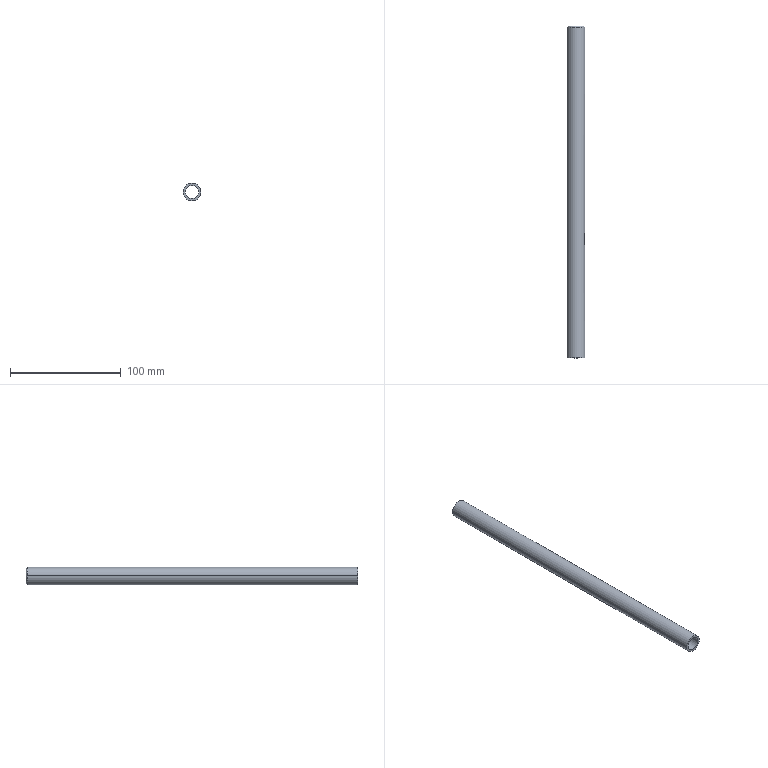Component | SolidWorks | GbgbMagnetPlacementTubeF8-1 | 1 solid | 11 faces | box 16 x 300 x 16 mm | volume 26347 mm3 | plane 5 | cylinder 4 | cone 2 | commonest cylinder face diameters 12 x2 16 x2
build123d program:
from build123d import *

# Parameters (mm, degrees)
SKETCH1_R           = 8
SKETCH1_R_2         = 6
BOSS_EXTRUDE1_DEPTH = 150
CHAMFER1_SIZE       = 1
SKETCH9_W           = 0.5
SKETCH9_H           = 10
CUT_EXTRUDE6_DEPTH  = 5


with BuildPart() as part:
    # Sketch1 → Boss-Extrude1 (new, symmetric)
    with BuildSketch(Plane(origin=(0, 0, 0), x_dir=(1, 0, 0), z_dir=(0, 1, 0))):
        with Locations(Location((0, 0, 0), (0, 0, 270))):
            Circle(SKETCH1_R)
        with Locations(Location((0, 0, 0), (0, 0, 270))):
            Circle(SKETCH1_R_2, mode=Mode.SUBTRACT)
    extrude(amount=BOSS_EXTRUDE1_DEPTH, both=True)

    # Chamfer1
    chamfer1_edges = [part.edges().sort_by_distance(p)[0] for p in [
        (0, -150, -8),
    ]]
    chamfer(chamfer1_edges, length=CHAMFER1_SIZE)

    # Sketch9 → Cut-Extrude6 (cut, symmetric)
    with BuildSketch(Plane(origin=(0, 0, 0), x_dir=(0, 0, -1), z_dir=(1, 0, 0))):
        with Locations((7.75, 42.5)):
            Rectangle(SKETCH9_W, SKETCH9_H)
    extrude(amount=CUT_EXTRUDE6_DEPTH, both=True, mode=Mode.SUBTRACT)


solid = part.part

# Placed as in the assembly
solid = solid.moved(Location((80.446, 537.34, 408.232), (180, -90, 0)))
STEP:
#1=COLOUR_RGB('',0.7922,0.8196,0.9333);
#2=FILL_AREA_STYLE_COLOUR('',#1);
#3=FILL_AREA_STYLE('',(#2));
#4=SURFACE_STYLE_FILL_AREA(#3);
#5=SURFACE_SIDE_STYLE('',(#4));
#6=SURFACE_STYLE_USAGE(.BOTH.,#5);
#7=PRESENTATION_STYLE_ASSIGNMENT((#6));
#8=CARTESIAN_POINT('',(3.443,27.061,16.072));
#9=VERTEX_POINT('',#8);
#10=CARTESIAN_POINT('',(2.892,27.061,16.072));
#11=VERTEX_POINT('',#10);
#12=CARTESIAN_POINT('',(3.167,27.061,16.072));
#13=DIRECTION('',(0.,1.,0.));
#14=DIRECTION('',(-1.,0.,0.));
#15=AXIS2_PLACEMENT_3D('',#12,#13,#14);
#16=CIRCLE('',#15,0.2756);
#17=EDGE_CURVE('',#9,#11,#16,.T.);
#18=ORIENTED_EDGE('',*,*,#17,.F.);
#19=CARTESIAN_POINT('',(3.482,27.021,16.072));
#20=VERTEX_POINT('',#19);
#21=CARTESIAN_POINT('',(3.482,27.021,16.072));
#22=DIRECTION('',(0.7071,-0.7071,-0.));
#23=VECTOR('',#22,39.37);
#24=LINE('',#21,#23);
#25=EDGE_CURVE('',#9,#20,#24,.T.);
#26=ORIENTED_EDGE('',*,*,#25,.T.);
#27=CARTESIAN_POINT('',(2.852,27.021,16.072));
#28=VERTEX_POINT('',#27);
#29=CARTESIAN_POINT('',(3.167,27.021,16.072));
#30=DIRECTION('',(-0.,-1.,-0.));
#31=DIRECTION('',(-1.,0.,0.));
#32=AXIS2_PLACEMENT_3D('',#29,#30,#31);
#33=CIRCLE('',#32,0.315);
#34=EDGE_CURVE('',#28,#20,#33,.T.);
#35=ORIENTED_EDGE('',*,*,#34,.F.);
#36=CARTESIAN_POINT('',(2.852,27.021,16.072));
#37=DIRECTION('',(-0.7071,-0.7071,-0.));
#38=VECTOR('',#37,39.37);
#39=LINE('',#36,#38);
#40=EDGE_CURVE('',#11,#28,#39,.T.);
#41=ORIENTED_EDGE('',*,*,#40,.F.);
#42=EDGE_LOOP('',(#18,#26,#35,#41));
#43=FACE_OUTER_BOUND('',#42,.T.);
#44=CARTESIAN_POINT('',(3.167,27.021,16.072));
#45=DIRECTION('',(-0.,-1.,-0.));
#46=DIRECTION('',(-1.,0.,0.));
#47=AXIS2_PLACEMENT_3D('',#44,#45,#46);
#48=CONICAL_SURFACE('',#47,0.315,0.7854);
#49=ADVANCED_FACE('',(#43),#48,.T.);
#50=CARTESIAN_POINT('',(3.403,15.25,16.072));
#51=VERTEX_POINT('',#50);
#52=CARTESIAN_POINT('',(2.931,15.25,16.072));
#53=VERTEX_POINT('',#52);
#54=CARTESIAN_POINT('',(3.167,15.25,16.072));
#55=DIRECTION('',(-0.,-1.,-0.));
#56=DIRECTION('',(-1.,0.,0.));
#57=AXIS2_PLACEMENT_3D('',#54,#55,#56);
#58=CIRCLE('',#57,0.2362);
#59=EDGE_CURVE('',#51,#53,#58,.T.);
#60=ORIENTED_EDGE('',*,*,#59,.T.);
#61=CARTESIAN_POINT('',(2.931,27.061,16.072));
#62=VERTEX_POINT('',#61);
#63=CARTESIAN_POINT('',(2.931,15.25,16.072));
#64=DIRECTION('',(0.,1.,0.));
#65=VECTOR('',#64,39.37);
#66=LINE('',#63,#65);
#67=EDGE_CURVE('',#53,#62,#66,.T.);
#68=ORIENTED_EDGE('',*,*,#67,.T.);
#69=CARTESIAN_POINT('',(3.403,27.061,16.072));
#70=VERTEX_POINT('',#69);
#71=CARTESIAN_POINT('',(3.167,27.061,16.072));
#72=DIRECTION('',(-0.,-1.,-0.));
#73=DIRECTION('',(-1.,0.,0.));
#74=AXIS2_PLACEMENT_3D('',#71,#72,#73);
#75=CIRCLE('',#74,0.2362);
#76=EDGE_CURVE('',#70,#62,#75,.T.);
#77=ORIENTED_EDGE('',*,*,#76,.F.);
#78=CARTESIAN_POINT('',(3.403,15.25,16.072));
#79=DIRECTION('',(0.,1.,0.));
#80=VECTOR('',#79,39.37);
#81=LINE('',#78,#80);
#82=EDGE_CURVE('',#51,#70,#81,.T.);
#83=ORIENTED_EDGE('',*,*,#82,.F.);
#84=EDGE_LOOP('',(#60,#68,#77,#83));
#85=FACE_OUTER_BOUND('',#84,.T.);
#86=CARTESIAN_POINT('',(3.167,15.25,16.072));
#87=DIRECTION('',(0.,1.,0.));
#88=DIRECTION('',(1.,0.,0.));
#89=AXIS2_PLACEMENT_3D('',#86,#87,#88);
#90=CYLINDRICAL_SURFACE('',#89,0.2362);
#91=ADVANCED_FACE('',(#85),#90,.F.);
#92=CARTESIAN_POINT('',(2.852,15.25,16.072));
#93=VERTEX_POINT('',#92);
#94=CARTESIAN_POINT('',(3.482,15.25,16.072));
#95=VERTEX_POINT('',#94);
#96=CARTESIAN_POINT('',(3.167,15.25,16.072));
#97=DIRECTION('',(-0.,-1.,-0.));
#98=DIRECTION('',(-1.,0.,0.));
#99=AXIS2_PLACEMENT_3D('',#96,#97,#98);
#100=CIRCLE('',#99,0.315);
#101=EDGE_CURVE('',#93,#95,#100,.T.);
#102=ORIENTED_EDGE('',*,*,#101,.F.);
#103=CARTESIAN_POINT('',(2.852,15.25,16.072));
#104=DIRECTION('',(0.,1.,0.));
#105=VECTOR('',#104,39.37);
#106=LINE('',#103,#105);
#107=EDGE_CURVE('',#93,#28,#106,.T.);
#108=ORIENTED_EDGE('',*,*,#107,.T.);
#109=ORIENTED_EDGE('',*,*,#34,.T.);
#110=CARTESIAN_POINT('',(3.482,19.679,16.072));
#111=VERTEX_POINT('',#110);
#112=CARTESIAN_POINT('',(3.482,15.25,16.072));
#113=DIRECTION('',(0.,1.,0.));
#114=VECTOR('',#113,39.37);
#115=LINE('',#112,#114);
#116=EDGE_CURVE('',#111,#20,#115,.T.);
#117=ORIENTED_EDGE('',*,*,#116,.F.);
#118=CARTESIAN_POINT('',(3.462,19.679,15.963));
#119=VERTEX_POINT('',#118);
#120=CARTESIAN_POINT('',(3.167,19.679,16.072));
#121=DIRECTION('',(0.,1.,0.));
#122=DIRECTION('',(1.,0.,0.));
#123=AXIS2_PLACEMENT_3D('',#120,#121,#122);
#124=CIRCLE('',#123,0.315);
#125=EDGE_CURVE('',#111,#119,#124,.T.);
#126=ORIENTED_EDGE('',*,*,#125,.T.);
#127=CARTESIAN_POINT('',(3.462,19.285,15.963));
#128=VERTEX_POINT('',#127);
#129=CARTESIAN_POINT('',(3.462,15.25,15.963));
#130=DIRECTION('',(-0.,-1.,-0.));
#131=VECTOR('',#130,39.37);
#132=LINE('',#129,#131);
#133=EDGE_CURVE('',#119,#128,#132,.T.);
#134=ORIENTED_EDGE('',*,*,#133,.T.);
#135=CARTESIAN_POINT('',(3.482,19.285,16.072));
#136=VERTEX_POINT('',#135);
#137=CARTESIAN_POINT('',(3.167,19.285,16.072));
#138=DIRECTION('',(-0.,-1.,-0.));
#139=DIRECTION('',(-1.,0.,0.));
#140=AXIS2_PLACEMENT_3D('',#137,#138,#139);
#141=CIRCLE('',#140,0.315);
#142=EDGE_CURVE('',#128,#136,#141,.T.);
#143=ORIENTED_EDGE('',*,*,#142,.T.);
#144=CARTESIAN_POINT('',(3.482,15.25,16.072));
#145=DIRECTION('',(0.,1.,0.));
#146=VECTOR('',#145,39.37);
#147=LINE('',#144,#146);
#148=EDGE_CURVE('',#95,#136,#147,.T.);
#149=ORIENTED_EDGE('',*,*,#148,.F.);
#150=EDGE_LOOP('',(#102,#108,#109,#117,#126,#134,#143,#149));
#151=FACE_OUTER_BOUND('',#150,.T.);
#152=CARTESIAN_POINT('',(3.167,15.25,16.072));
#153=DIRECTION('',(0.,1.,0.));
#154=DIRECTION('',(1.,0.,0.));
#155=AXIS2_PLACEMENT_3D('',#152,#153,#154);
#156=CYLINDRICAL_SURFACE('',#155,0.315);
#157=ADVANCED_FACE('',(#151),#156,.T.);
#158=CARTESIAN_POINT('',(3.167,15.25,16.072));
#159=DIRECTION('',(-0.,-1.,-0.));
#160=DIRECTION('',(-1.,0.,0.));
#161=AXIS2_PLACEMENT_3D('',#158,#159,#160);
#162=CIRCLE('',#161,0.315);
#163=EDGE_CURVE('',#95,#93,#162,.T.);
#164=ORIENTED_EDGE('',*,*,#163,.T.);
#165=ORIENTED_EDGE('',*,*,#101,.T.);
#166=EDGE_LOOP('',(#164,#165));
#167=FACE_OUTER_BOUND('',#166,.T.);
#168=ORIENTED_EDGE('',*,*,#59,.F.);
#169=CARTESIAN_POINT('',(3.167,15.25,16.072));
#170=DIRECTION('',(-0.,-1.,-0.));
#171=DIRECTION('',(-1.,0.,0.));
#172=AXIS2_PLACEMENT_3D('',#169,#170,#171);
#173=CIRCLE('',#172,0.2362);
#174=EDGE_CURVE('',#53,#51,#173,.T.);
#175=ORIENTED_EDGE('',*,*,#174,.F.);
#176=EDGE_LOOP('',(#168,#175));
#177=FACE_BOUND('',#176,.T.);
#178=CARTESIAN_POINT('',(3.167,15.25,16.072));
#179=DIRECTION('',(-0.,-1.,-0.));
#180=DIRECTION('',(-1.,0.,0.));
#181=AXIS2_PLACEMENT_3D('',#178,#179,#180);
#182=PLANE('',#181);
#183=ADVANCED_FACE('',(#167,#177),#182,.T.);
#184=CARTESIAN_POINT('',(3.167,27.061,16.072));
#185=DIRECTION('',(0.,1.,0.));
#186=DIRECTION('',(-1.,0.,0.));
#187=AXIS2_PLACEMENT_3D('',#184,#185,#186);
#188=CIRCLE('',#187,0.2756);
#189=EDGE_CURVE('',#11,#9,#188,.T.);
#190=ORIENTED_EDGE('',*,*,#189,.T.);
#191=ORIENTED_EDGE('',*,*,#17,.T.);
#192=EDGE_LOOP('',(#190,#191));
#193=FACE_OUTER_BOUND('',#192,.T.);
#194=ORIENTED_EDGE('',*,*,#76,.T.);
#195=CARTESIAN_POINT('',(3.167,27.061,16.072));
#196=DIRECTION('',(-0.,-1.,-0.));
#197=DIRECTION('',(-1.,0.,0.));
#198=AXIS2_PLACEMENT_3D('',#195,#196,#197);
#199=CIRCLE('',#198,0.2362);
#200=EDGE_CURVE('',#62,#70,#199,.T.);
#201=ORIENTED_EDGE('',*,*,#200,.T.);
#202=EDGE_LOOP('',(#194,#201));
#203=FACE_BOUND('',#202,.T.);
#204=CARTESIAN_POINT('',(3.167,27.061,16.072));
#205=DIRECTION('',(-0.,-1.,-0.));
#206=DIRECTION('',(-1.,0.,0.));
#207=AXIS2_PLACEMENT_3D('',#204,#205,#206);
#208=PLANE('',#207);
#209=ADVANCED_FACE('',(#193,#203),#208,.F.);
#210=ORIENTED_EDGE('',*,*,#107,.F.);
#211=ORIENTED_EDGE('',*,*,#163,.F.);
#212=ORIENTED_EDGE('',*,*,#148,.T.);
#213=CARTESIAN_POINT('',(3.462,19.285,16.182));
#214=VERTEX_POINT('',#213);
#215=CARTESIAN_POINT('',(3.167,19.285,16.072));
#216=DIRECTION('',(-0.,-1.,-0.));
#217=DIRECTION('',(-1.,0.,0.));
#218=AXIS2_PLACEMENT_3D('',#215,#216,#217);
#219=CIRCLE('',#218,0.315);
#220=EDGE_CURVE('',#136,#214,#219,.T.);
#221=ORIENTED_EDGE('',*,*,#220,.T.);
#222=CARTESIAN_POINT('',(3.462,19.679,16.182));
#223=VERTEX_POINT('',#222);
#224=CARTESIAN_POINT('',(3.462,15.25,16.182));
#225=DIRECTION('',(0.,1.,0.));
#226=VECTOR('',#225,39.37);
#227=LINE('',#224,#226);
#228=EDGE_CURVE('',#214,#223,#227,.T.);
#229=ORIENTED_EDGE('',*,*,#228,.T.);
#230=CARTESIAN_POINT('',(3.167,19.679,16.072));
#231=DIRECTION('',(0.,1.,0.));
#232=DIRECTION('',(1.,0.,0.));
#233=AXIS2_PLACEMENT_3D('',#230,#231,#232);
#234=CIRCLE('',#233,0.315);
#235=EDGE_CURVE('',#223,#111,#234,.T.);
#236=ORIENTED_EDGE('',*,*,#235,.T.);
#237=ORIENTED_EDGE('',*,*,#116,.T.);
#238=CARTESIAN_POINT('',(3.167,27.021,16.072));
#239=DIRECTION('',(-0.,-1.,-0.));
#240=DIRECTION('',(-1.,0.,0.));
#241=AXIS2_PLACEMENT_3D('',#238,#239,#240);
#242=CIRCLE('',#241,0.315);
#243=EDGE_CURVE('',#20,#28,#242,.T.);
#244=ORIENTED_EDGE('',*,*,#243,.T.);
#245=EDGE_LOOP('',(#210,#211,#212,#221,#229,#236,#237,#244));
#246=FACE_OUTER_BOUND('',#245,.T.);
#247=CARTESIAN_POINT('',(3.167,15.25,16.072));
#248=DIRECTION('',(0.,1.,0.));
#249=DIRECTION('',(1.,0.,0.));
#250=AXIS2_PLACEMENT_3D('',#247,#248,#249);
#251=CYLINDRICAL_SURFACE('',#250,0.315);
#252=ADVANCED_FACE('',(#246),#251,.T.);
#253=ORIENTED_EDGE('',*,*,#67,.F.);
#254=ORIENTED_EDGE('',*,*,#174,.T.);
#255=ORIENTED_EDGE('',*,*,#82,.T.);
#256=ORIENTED_EDGE('',*,*,#200,.F.);
#257=EDGE_LOOP('',(#253,#254,#255,#256));
#258=FACE_OUTER_BOUND('',#257,.T.);
#259=CARTESIAN_POINT('',(3.167,15.25,16.072));
#260=DIRECTION('',(0.,1.,0.));
#261=DIRECTION('',(1.,0.,0.));
#262=AXIS2_PLACEMENT_3D('',#259,#260,#261);
#263=CYLINDRICAL_SURFACE('',#262,0.2362);
#264=ADVANCED_FACE('',(#258),#263,.F.);
#265=ORIENTED_EDGE('',*,*,#25,.F.);
#266=ORIENTED_EDGE('',*,*,#189,.F.);
#267=ORIENTED_EDGE('',*,*,#40,.T.);
#268=ORIENTED_EDGE('',*,*,#243,.F.);
#269=EDGE_LOOP('',(#265,#266,#267,#268));
#270=FACE_OUTER_BOUND('',#269,.T.);
#271=CARTESIAN_POINT('',(3.167,27.021,16.072));
#272=DIRECTION('',(-0.,-1.,-0.));
#273=DIRECTION('',(-1.,0.,0.));
#274=AXIS2_PLACEMENT_3D('',#271,#272,#273);
#275=CONICAL_SURFACE('',#274,0.315,0.7854);
#276=ADVANCED_FACE('',(#270),#275,.T.);
#277=ORIENTED_EDGE('',*,*,#235,.F.);
#278=CARTESIAN_POINT('',(3.462,19.679,16.269));
#279=DIRECTION('',(-0.,0.,-1.));
#280=VECTOR('',#279,39.37);
#281=LINE('',#278,#280);
#282=EDGE_CURVE('',#223,#119,#281,.T.);
#283=ORIENTED_EDGE('',*,*,#282,.T.);
#284=ORIENTED_EDGE('',*,*,#125,.F.);
#285=EDGE_LOOP('',(#277,#283,#284));
#286=FACE_OUTER_BOUND('',#285,.T.);
#287=CARTESIAN_POINT('',(3.482,19.679,16.269));
#288=DIRECTION('',(0.,1.,0.));
#289=DIRECTION('',(1.,-0.,-0.));
#290=AXIS2_PLACEMENT_3D('',#287,#288,#289);
#291=PLANE('',#290);
#292=ADVANCED_FACE('',(#286),#291,.F.);
#293=CARTESIAN_POINT('',(3.462,19.285,16.269));
#294=DIRECTION('',(-0.,0.,-1.));
#295=VECTOR('',#294,39.37);
#296=LINE('',#293,#295);
#297=EDGE_CURVE('',#214,#128,#296,.T.);
#298=ORIENTED_EDGE('',*,*,#297,.T.);
#299=ORIENTED_EDGE('',*,*,#133,.F.);
#300=ORIENTED_EDGE('',*,*,#282,.F.);
#301=ORIENTED_EDGE('',*,*,#228,.F.);
#302=EDGE_LOOP('',(#298,#299,#300,#301));
#303=FACE_OUTER_BOUND('',#302,.T.);
#304=CARTESIAN_POINT('',(3.462,19.679,16.269));
#305=DIRECTION('',(-1.,0.,0.));
#306=DIRECTION('',(-0.,0.,-1.));
#307=AXIS2_PLACEMENT_3D('',#304,#305,#306);
#308=PLANE('',#307);
#309=ADVANCED_FACE('',(#303),#308,.F.);
#310=ORIENTED_EDGE('',*,*,#297,.F.);
#311=ORIENTED_EDGE('',*,*,#220,.F.);
#312=ORIENTED_EDGE('',*,*,#142,.F.);
#313=EDGE_LOOP('',(#310,#311,#312));
#314=FACE_OUTER_BOUND('',#313,.T.);
#315=CARTESIAN_POINT('',(3.482,19.285,16.269));
#316=DIRECTION('',(-0.,-1.,-0.));
#317=DIRECTION('',(-1.,0.,0.));
#318=AXIS2_PLACEMENT_3D('',#315,#316,#317);
#319=PLANE('',#318);
#320=ADVANCED_FACE('',(#314),#319,.F.);
#321=CLOSED_SHELL('',(#49,#91,#157,#183,#209,#252,#264,#276,#292,#309,#320));
#322=MANIFOLD_SOLID_BREP('',#321);
#323=STYLED_ITEM('',(#7),#322);
#324=PRESENTATION_LAYER_ASSIGNMENT('','',(#323));
#325=(LENGTH_UNIT()NAMED_UNIT(*)SI_UNIT($,.METRE.));
#326=LENGTH_MEASURE_WITH_UNIT(LENGTH_MEASURE(0.0254),#325);
#327=DIMENSIONAL_EXPONENTS(1.,0.,0.,0.,0.,0.,0.);
#328=(CONVERSION_BASED_UNIT('',#326)LENGTH_UNIT()NAMED_UNIT(#327));
#329=UNCERTAINTY_MEASURE_WITH_UNIT(LENGTH_MEASURE(0.00001),#328,'','');
#330=(NAMED_UNIT(*)PLANE_ANGLE_UNIT()SI_UNIT($,.RADIAN.));
#331=(NAMED_UNIT(*)SI_UNIT($,.STERADIAN.)SOLID_ANGLE_UNIT());
#332=(GEOMETRIC_REPRESENTATION_CONTEXT(3)GLOBAL_UNCERTAINTY_ASSIGNED_CONTEXT((#329))GLOBAL_UNIT_ASSIGNED_CONTEXT((#328,#330,#331))REPRESENTATION_CONTEXT('',''));
#333=MECHANICAL_DESIGN_GEOMETRIC_PRESENTATION_REPRESENTATION('',(#323),#332);
#334=CARTESIAN_POINT('',(0.,0.,0.));
#335=DIRECTION('',(0.,0.,1.));
#336=DIRECTION('',(1.,0.,0.));
#337=AXIS2_PLACEMENT_3D('',#334,#335,#336);
#338=(LENGTH_UNIT()NAMED_UNIT(*)SI_UNIT($,.METRE.));
#339=LENGTH_MEASURE_WITH_UNIT(LENGTH_MEASURE(0.0254),#338);
#340=DIMENSIONAL_EXPONENTS(1.,0.,0.,0.,0.,0.,0.);
#341=(CONVERSION_BASED_UNIT('',#339)LENGTH_UNIT()NAMED_UNIT(#340));
#342=UNCERTAINTY_MEASURE_WITH_UNIT(LENGTH_MEASURE(0.00001),#341,'','');
#343=(NAMED_UNIT(*)PLANE_ANGLE_UNIT()SI_UNIT($,.RADIAN.));
#344=(NAMED_UNIT(*)SI_UNIT($,.STERADIAN.)SOLID_ANGLE_UNIT());
#345=(GEOMETRIC_REPRESENTATION_CONTEXT(3)GLOBAL_UNCERTAINTY_ASSIGNED_CONTEXT((#342))GLOBAL_UNIT_ASSIGNED_CONTEXT((#341,#343,#344))REPRESENTATION_CONTEXT('',''));
#346=ADVANCED_BREP_SHAPE_REPRESENTATION('',(#322,#337),#345);